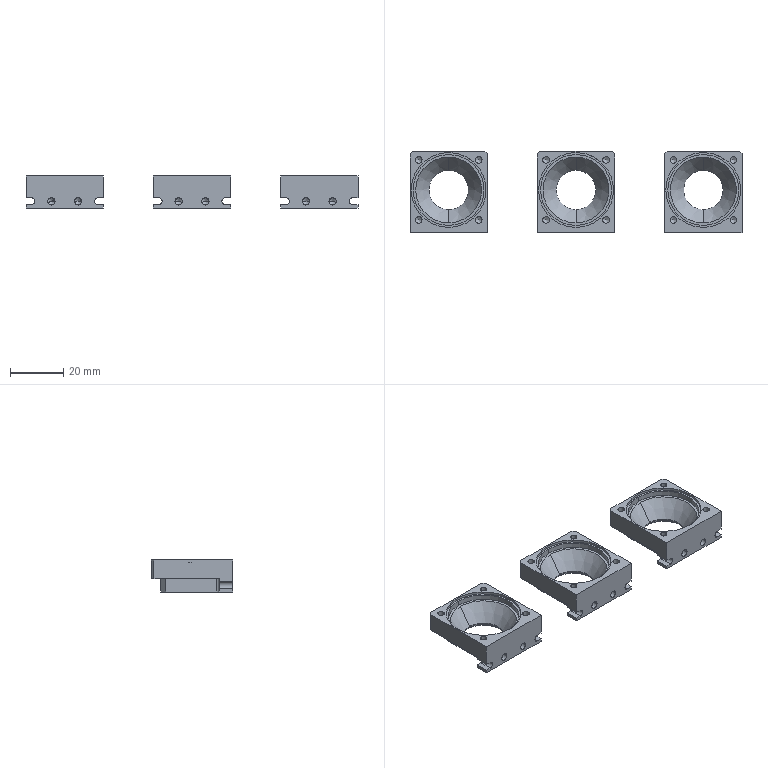CAM job | Mastercam | mm | 29 operations | part box 124.5 x 30.5 x 12
1. 3D High Speed (Dynamic OptiRough) | 11 - 10C
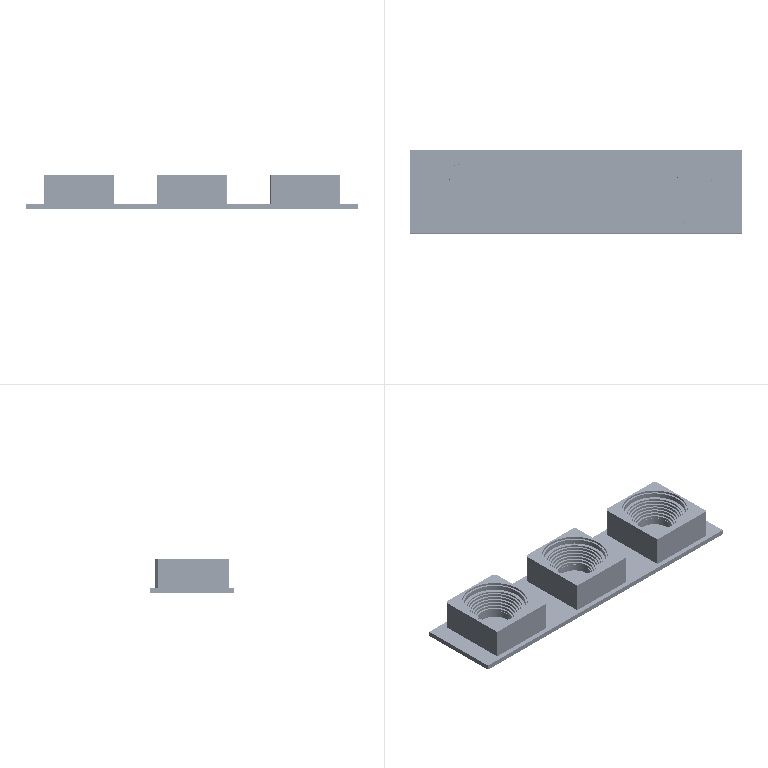2. Facing | 12 - 10J
3. Contour (2D) | 12 - 10J
4. Contour (2D) | 12 - 10J
5. Contour (2D) | 12 - 10J
6. Drill/Counterbore | 5 - 4 倒角刀
7. Peck Drill | 9 - 2.5 钻头
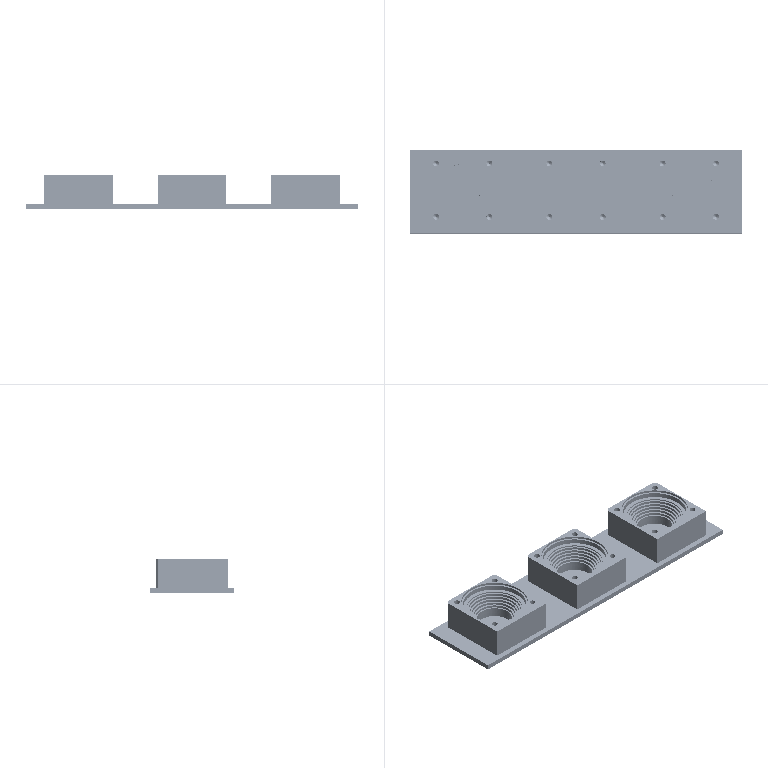8. Chamfer Drill | 5 - 4 倒角刀
9. Model Chamfer | 5 - 4 倒角刀
10. Model Chamfer | 5 - 4 倒角刀
11. Surface Finish Flowline | 16 - 8 圆鼻铣刀
12. Drill/Counterbore | 5 - 4 倒角刀
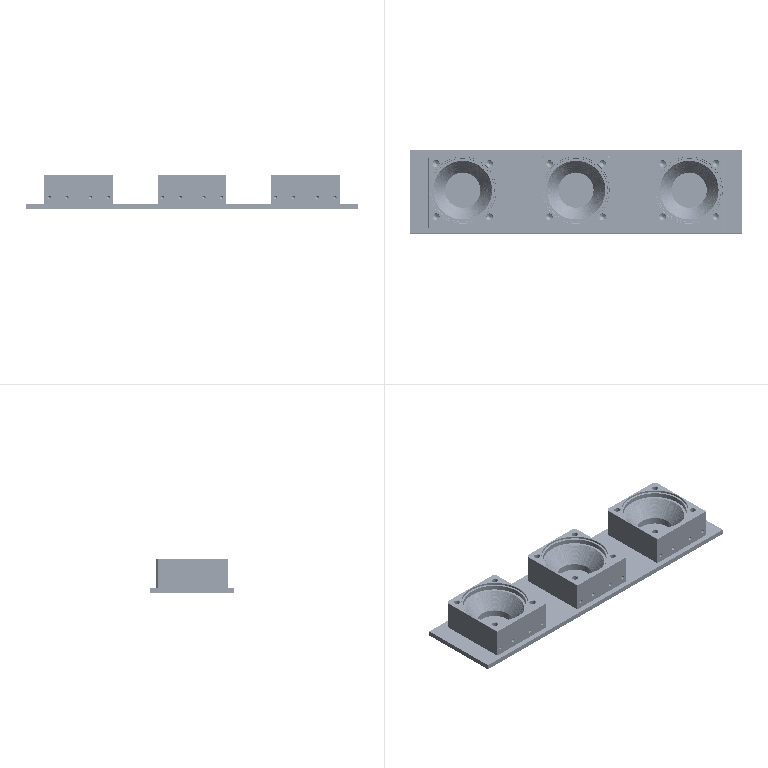13. Drill/Counterbore | 17 - 2.6 钻头
14. Contour (Ramp) | 3 - 2C
15. Contour (2D) | 4 - 2J
16. Contour (2D chamfer) | 5 - 4 倒角刀
17. Chamfer Drill | 5 - 4 倒角刀
18. Facing | 11 - 10C
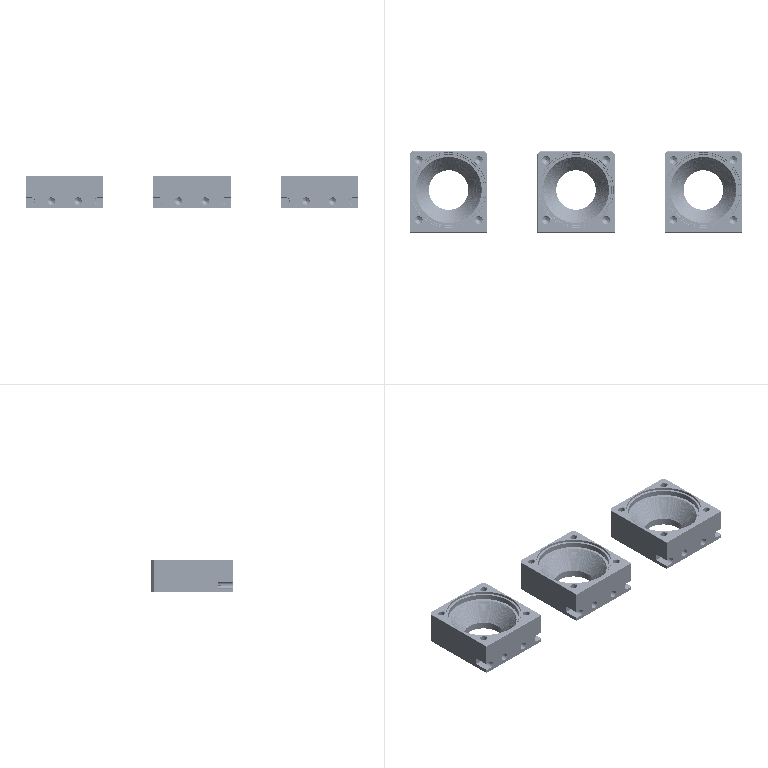19. 3D High Speed (Dynamic OptiRough) | 1 - 6C
20. Triangular mesh Triangular mesh | 2 - 6J
21. Contour (Remachining) | 6 - 4C
22. Contour (2D) | 7 - 4J
23. Contour (2D) | 7 - 4J
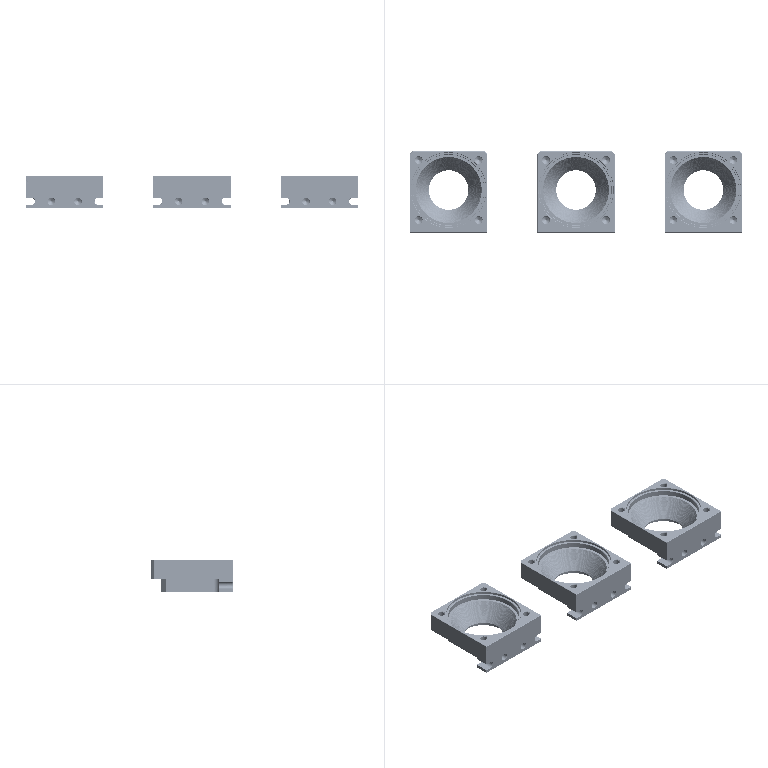24. Contour (Remachining) | 4 - 2J
25. Drill/Counterbore | 5 - 4 倒角刀
26. Peck Drill | 10 - 1.6 钻头
27. Chamfer Drill | 14 - 3 倒角刀
28. Model Chamfer | 14 - 3 倒角刀
29. Model Chamfer | 14 - 3 倒角刀